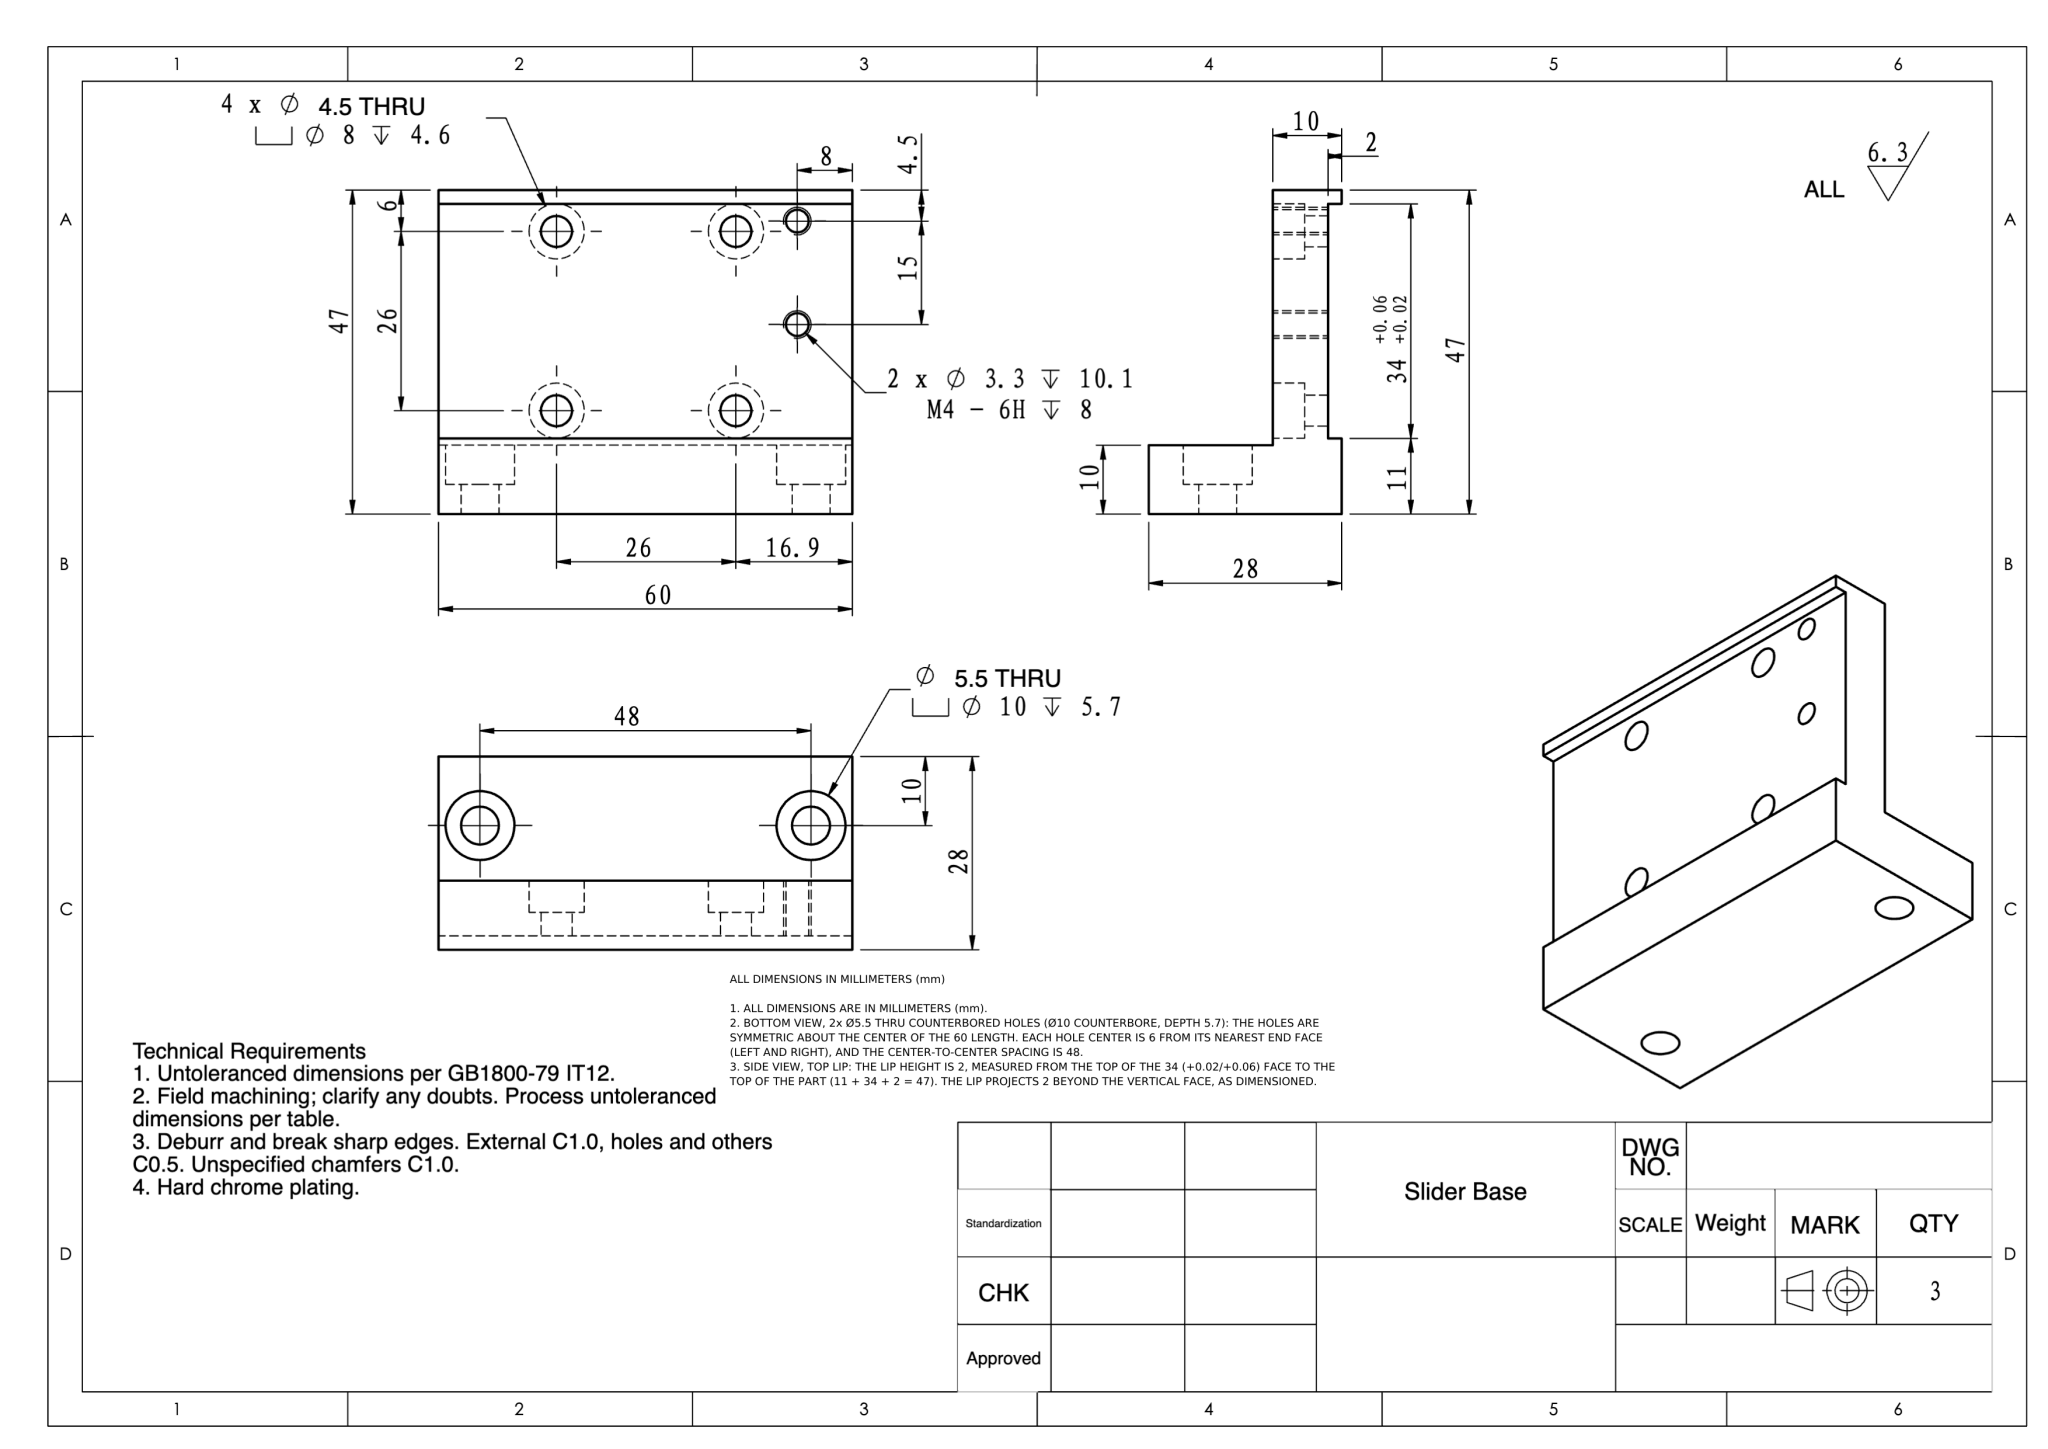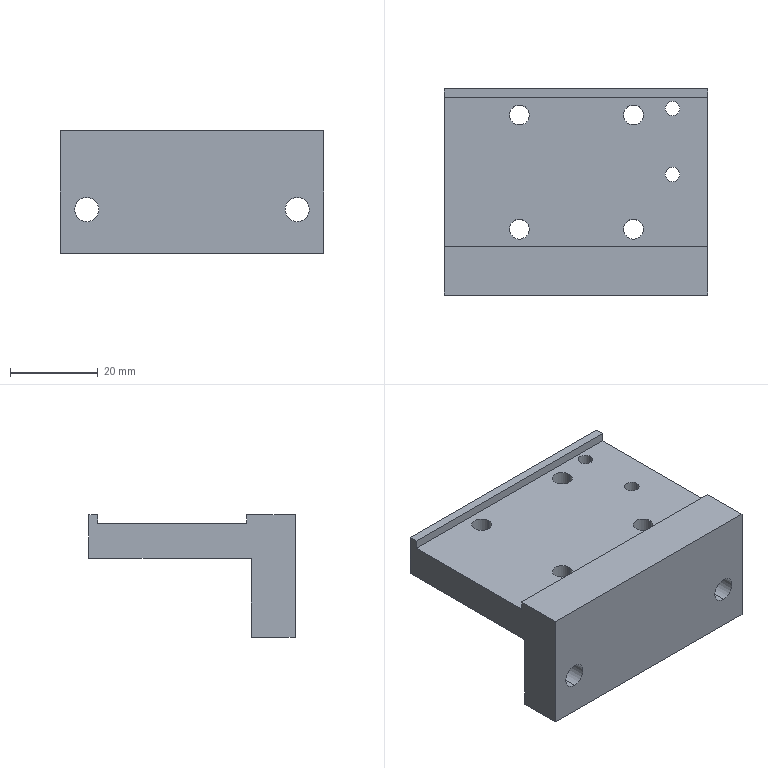Part | NX | mm | L-Shaped Slider Base | 1 solid | 46 faces | box 60 x 47 x 28 mm | volume 32542 mm3 | cylinder 28 | plane 18 | commonest cylinder face diameters 8 x8 4.5 x8 3.3 x4 10 x4 5.5 x4